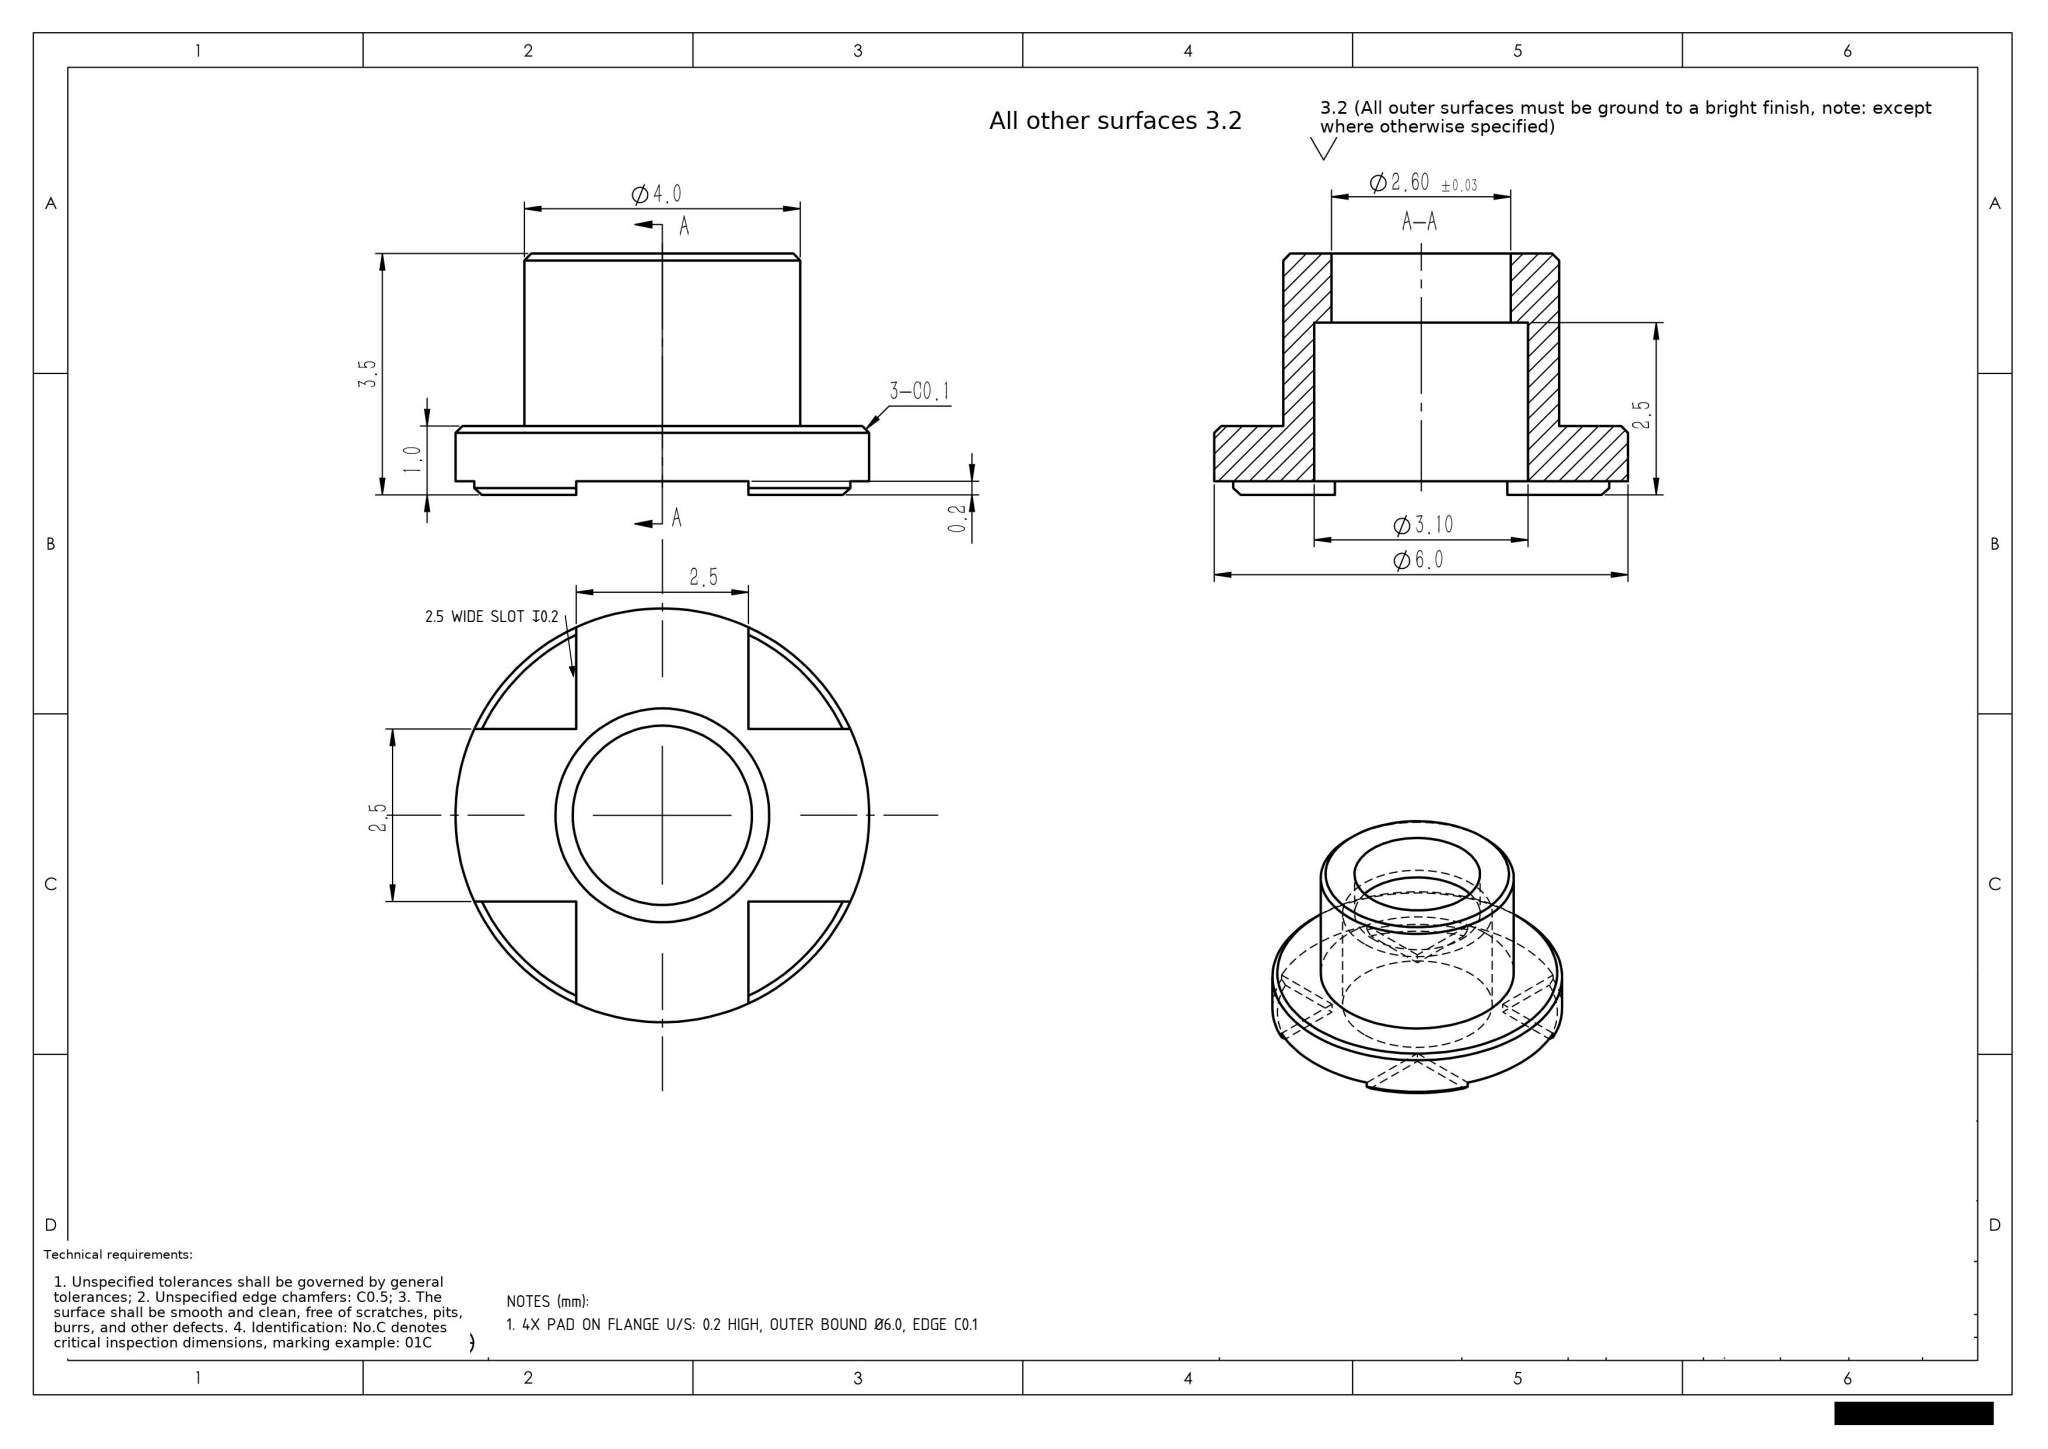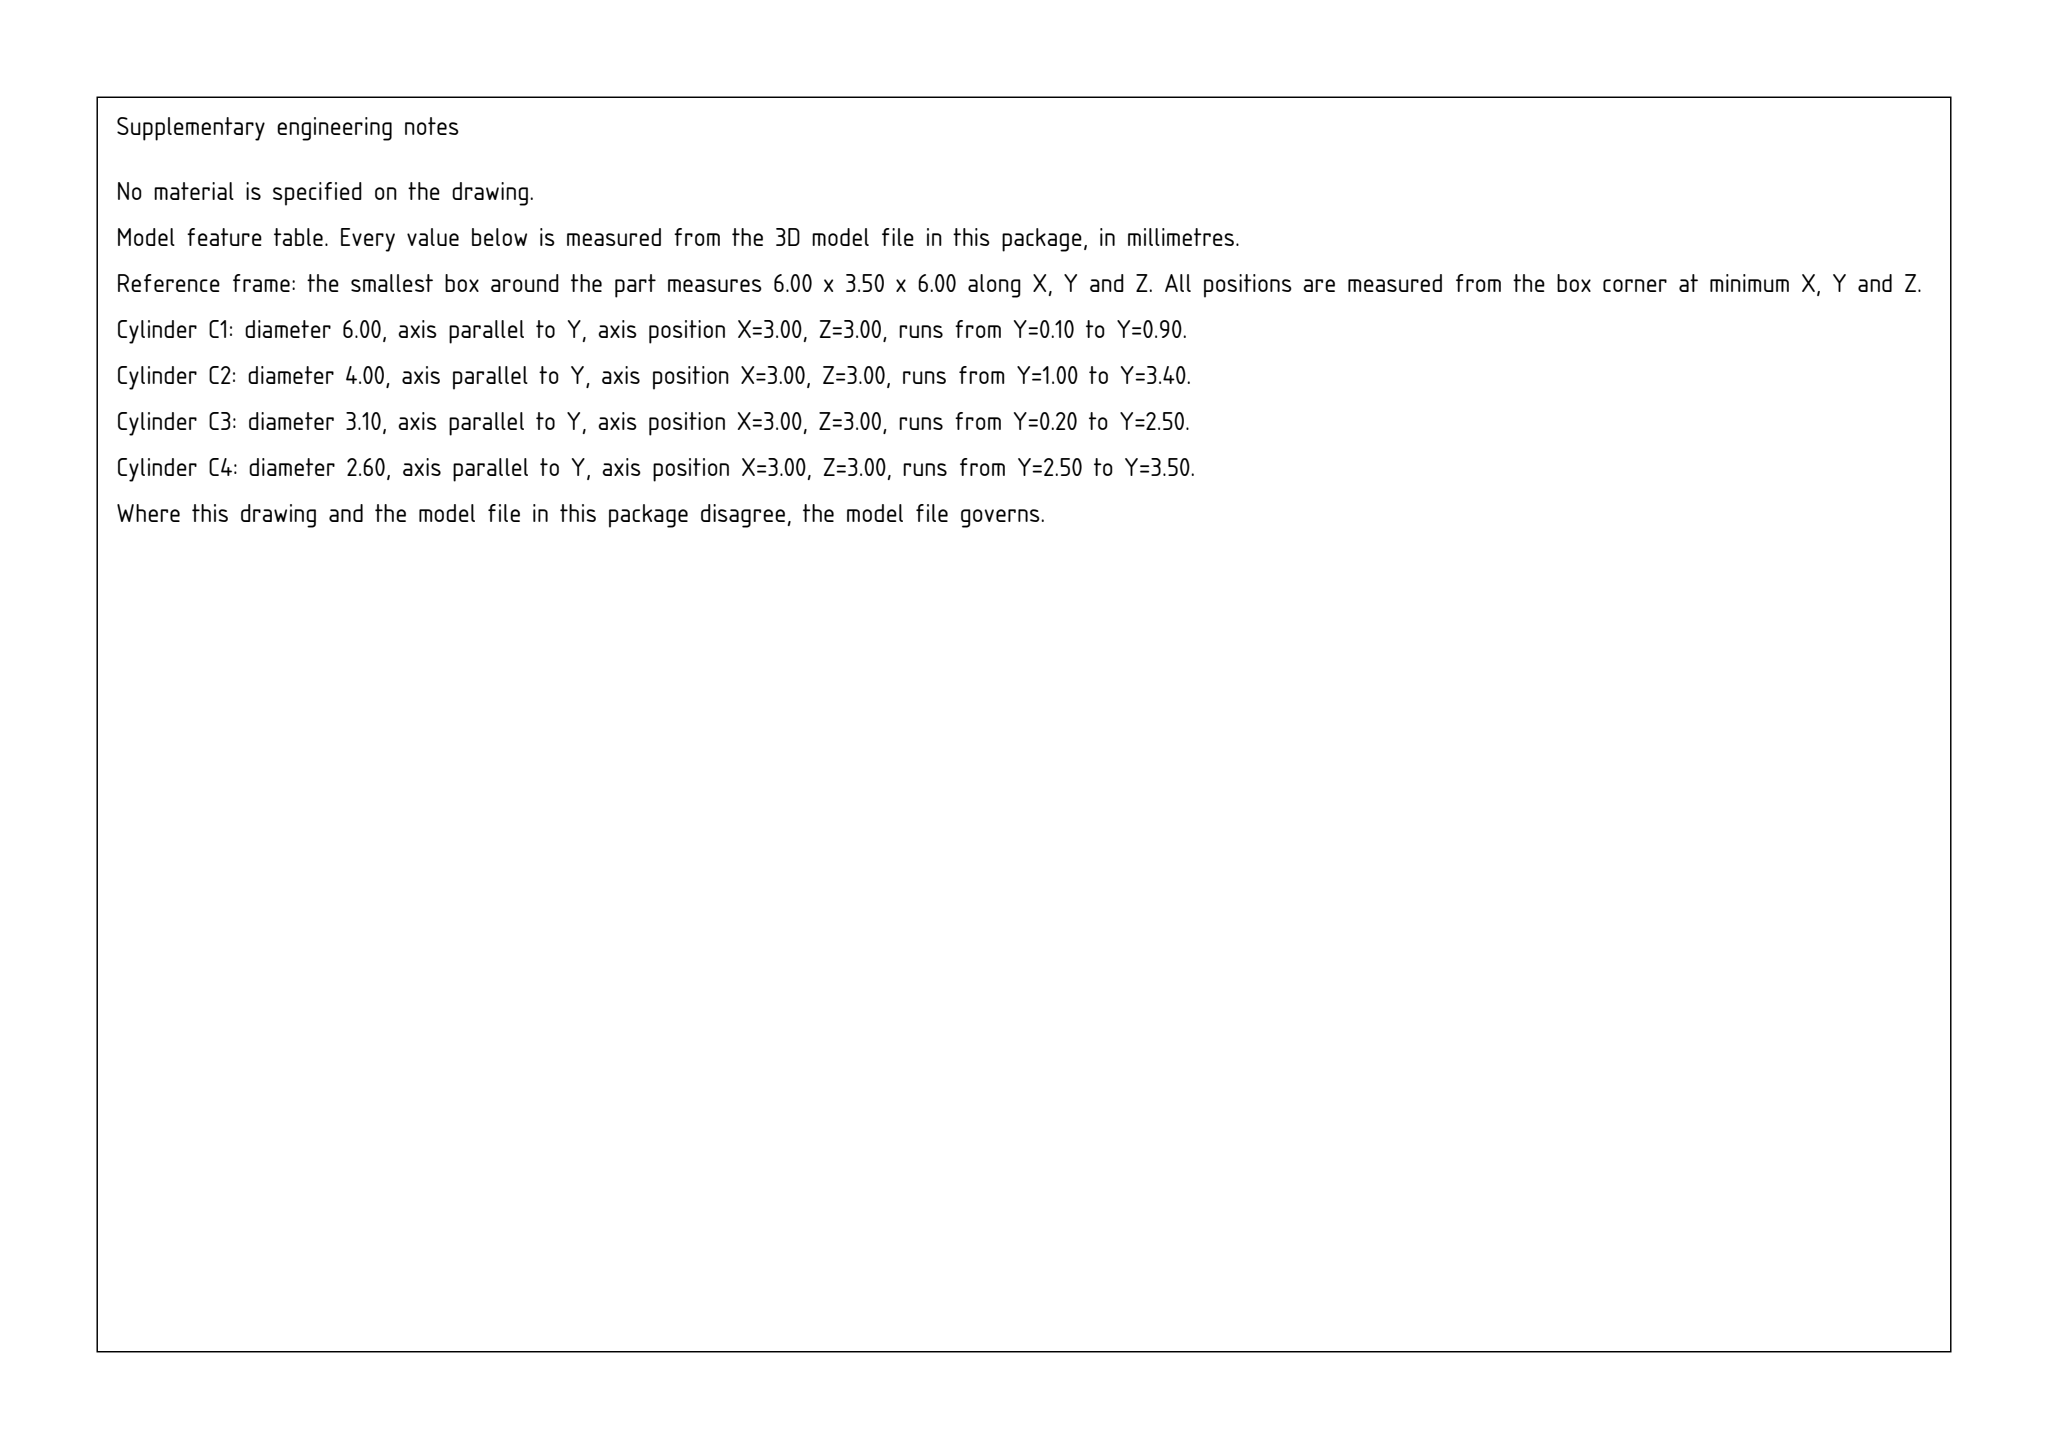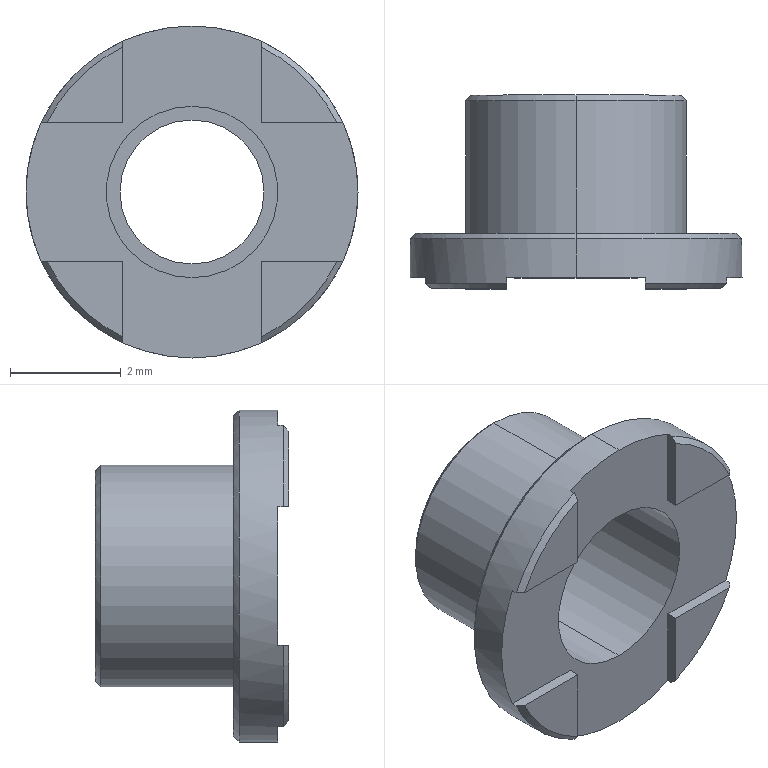Part | SolidWorks | mm | 1 solid | 32 faces | box 6 x 3.5 x 6 mm | volume 32 mm3 | plane 16 | cone 8 | cylinder 8 | commonest cylinder face diameters 2.6 x2 3.1 x2 4 x2 6 x2
Drawing notes:
FLANGE U/S CROSS RECESS: 2.5 WIDE SLOTS, 0.2 DEEP, OPEN TO Ø6.0 OD | from the solid: Walls at x=1.7 & 4.2 (and z=1.7 & 4.2), y 0-0.2; bottom face plane y=0.2 full Ø6.0; pad faces at y=0.0
4X PAD ON FLANGE U/S: 0.2 HIGH, OUTER BOUND Ø6.0, EDGE C0.1 | from the solid: 4X y=0 faces x[0.4,1.8]/[4.2,5.6] z[0.4,1.8]/[4.2,5.6]; 90° cones ref dia 5.8 at y=0; Ø6.0 flange
build123d program:
from build123d import *

# Parameters (mm, degrees)
SKETCH3_R          = 1.55
CUT_EXTRUDE2_DEPTH = 2.5
SKETCH4_R          = 1.3
CUT_EXTRUDE3_DEPTH = 6.5
CUT_EXTRUDE4_DEPTH = 0.2
CHAMFER1_SIZE      = 0.1


with BuildPart() as part:
    # Sketch1 → Revolve1 (revolve)
    with BuildSketch(Plane.XY, mode=Mode.PRIVATE) as revolve1_sk:
        Polygon((0, 0), (3, 0), (3, 1), (2, 1), (2, 3.5), (0, 3.5), align=None)
    revolve(revolve1_sk.sketch.rotate(Axis((0, 0, 0), (0, 1, 0)), 90), axis=Axis((0, 0, 0), (0, 1, 0)))

    # Sketch3 → Cut-Extrude2 (cut)
    with BuildSketch(Plane.XZ):
        with Locations(Location((0, 0, 0), (0, 0, 270))):
            Circle(SKETCH3_R)
    extrude(amount=-CUT_EXTRUDE2_DEPTH, mode=Mode.SUBTRACT)

    # Sketch4 → Cut-Extrude3 (cut, through all)
    with BuildSketch(Plane(origin=(0, 3.5, 0), x_dir=(1, 0, 0), z_dir=(0, 1, 0))):
        with Locations(Location((0, 0, 0), (0, 0, 270))):
            Circle(SKETCH4_R)
    extrude(amount=-CUT_EXTRUDE3_DEPTH, mode=Mode.SUBTRACT)

    # Sketch5 → Cut-Extrude4 (cut)
    with BuildSketch(Plane.XZ):
        Polygon((1.25, -1.25), (1.25, -3), (-1.25, -3), (-1.25, -1.25), (-3, -1.25), (-3, 1.25), (-1.25, 1.25), (-1.25, 3), (1.25, 3), (1.25, 1.25), (3, 1.25), (3, -1.25), align=None)
    extrude(amount=-CUT_EXTRUDE4_DEPTH, mode=Mode.SUBTRACT)

    # Chamfer1
    chamfer1_edges = [part.edges().sort_by_distance(p)[0] for p in [
        (2.121, 0, -2.121),
        (2.121, 0, 2.121),
        (-2.121, 0, 2.121),
        (-2.121, 0, -2.121),
        (0, 3.5, 2),
        (0, 1, 3),
    ]]
    chamfer(chamfer1_edges, length=CHAMFER1_SIZE)


solid = part.part